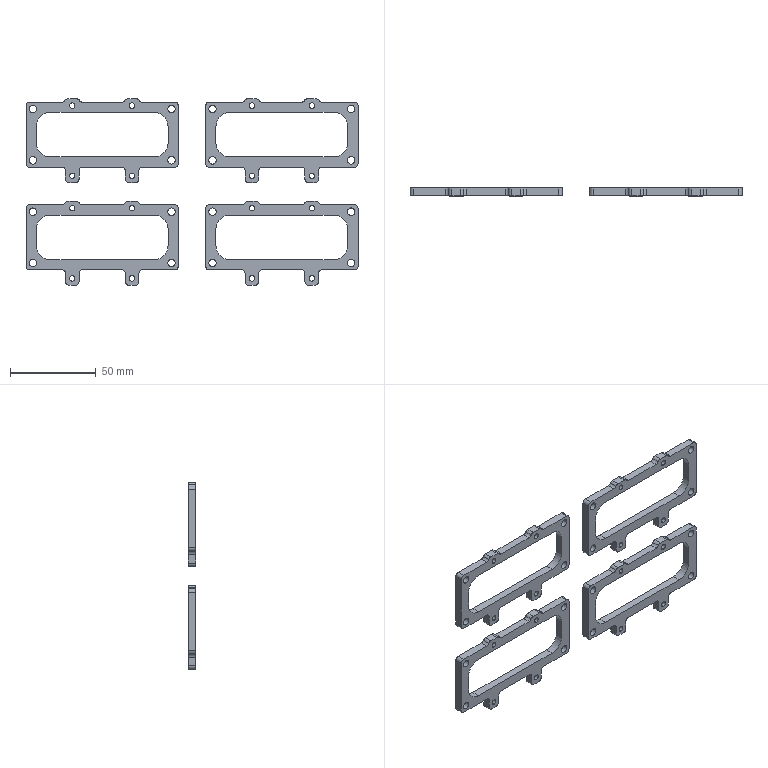CAM job | Mastercam | mm | 6 operations | part box 194 x 4.5 x 109
1. 2D High Speed (2D Area Mill) | 6 - 6 平铣刀
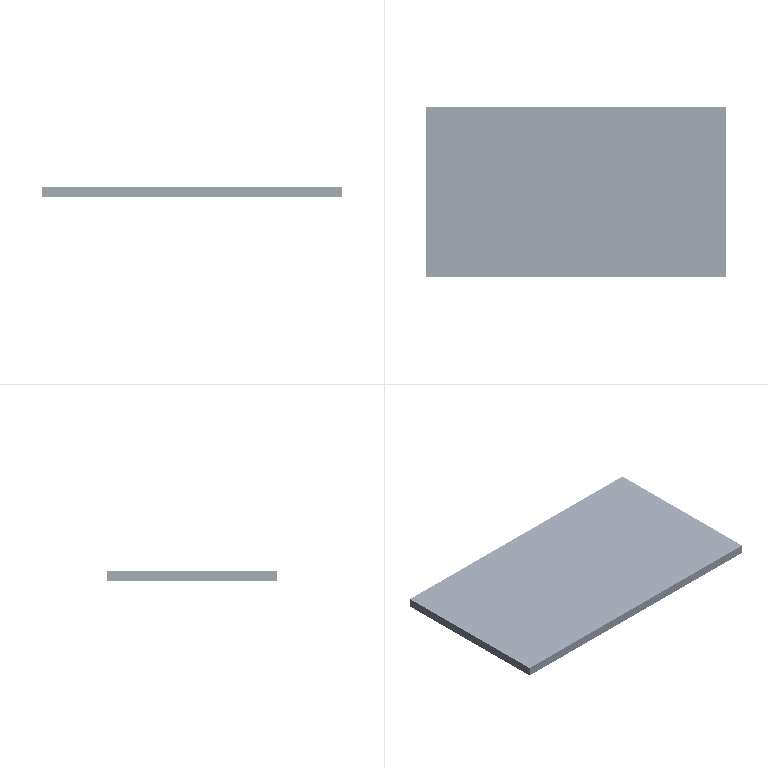2. Contour (2D chamfer) | 5 - 4 倒角刀
3. Helix Bore | 4 - 4 平铣刀
4. Contour (Ramp) | 4 - 4 平铣刀
5. Contour (Ramp) | 4 - 4 平铣刀
6. Drill/Counterbore | 5 - 4 倒角刀